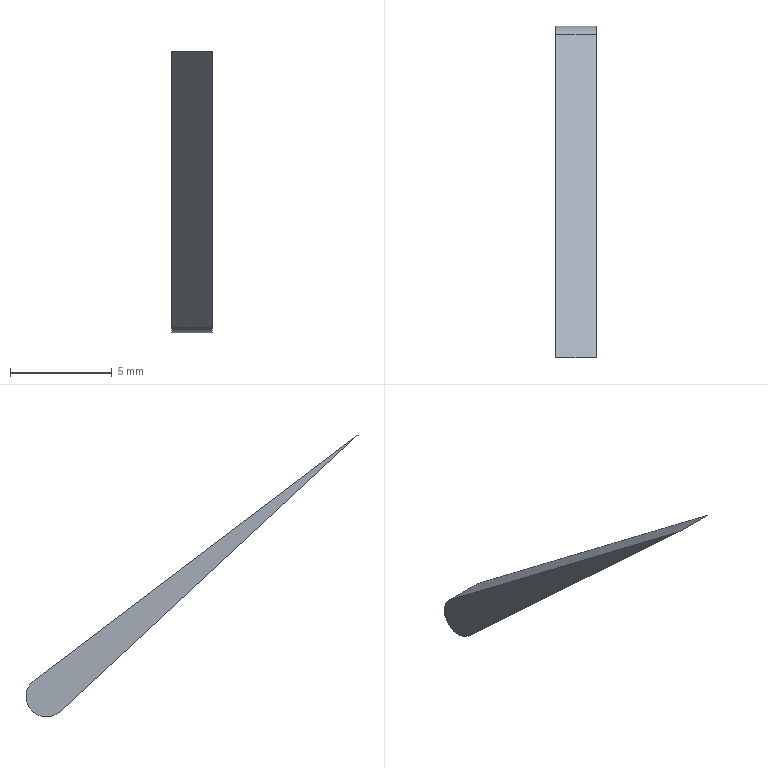Component | NX | SECONDHAND1 | 1 solid | 5 faces | box 2 x 16.32 x 13.86 mm | volume 43 mm3 | plane 4 | cylinder 1 | commonest cylinder face diameters 2 x1
STEP:
#1=CARTESIAN_POINT('',(0.,0.,0.));
#2=DIRECTION('',(0.,0.,1.));
#3=DIRECTION('',(1.,0.,0.));
#4=AXIS2_PLACEMENT_3D('',#1,#2,#3);
#5=CARTESIAN_POINT('',(-150.42,280.577,29.739));
#6=VERTEX_POINT('',#5);
#7=CARTESIAN_POINT('',(-150.42,281.861,31.269));
#8=VERTEX_POINT('',#7);
#9=CARTESIAN_POINT('',(-150.42,281.257,30.472));
#10=DIRECTION('',(1.,0.,0.));
#11=DIRECTION('',(0.,-0.766,0.6428));
#12=AXIS2_PLACEMENT_3D('',#9,#10,#11);
#13=CIRCLE('',#12,1.);
#14=CARTESIAN_POINT('',(-148.42,281.257,30.472));
#15=DIRECTION('',(-1.,0.,0.));
#16=DIRECTION('',(0.,0.766,-0.6428));
#17=AXIS2_PLACEMENT_3D('',#14,#15,#16);
#18=CYLINDRICAL_SURFACE('',#17,1.);
#19=CARTESIAN_POINT('',(9.425,2.));
#20=DIRECTION('',(-1.,0.));
#21=VECTOR('',#20,1.);
#22=LINE('',#19,#21);
#23=(GEOMETRIC_REPRESENTATION_CONTEXT(2)PARAMETRIC_REPRESENTATION_CONTEXT()REPRESENTATION_CONTEXT('',''));
#24=DEFINITIONAL_REPRESENTATION('',(#22),#23);
#25=PCURVE('',#18,#24);
#26=CARTESIAN_POINT('',(-150.42,281.257,30.472));
#27=DIRECTION('',(1.,0.,0.));
#28=DIRECTION('',(0.,-0.766,0.6428));
#29=AXIS2_PLACEMENT_3D('',#26,#27,#28);
#30=PLANE('',#29);
#31=CARTESIAN_POINT('',(0.,0.));
#32=DIRECTION('',(1.,-0.));
#33=AXIS2_PLACEMENT_2D('',#31,#32);
#34=CIRCLE('',#33,1.);
#35=(GEOMETRIC_REPRESENTATION_CONTEXT(2)PARAMETRIC_REPRESENTATION_CONTEXT()REPRESENTATION_CONTEXT('',''));
#36=DEFINITIONAL_REPRESENTATION('',(#34),#35);
#37=PCURVE('',#30,#36);
#38=SURFACE_CURVE('',#13,(#25,#37),.PCURVE_S1.);
#39=EDGE_CURVE('',#6,#8,#38,.T.);
#40=ORIENTED_EDGE('',*,*,#39,.T.);
#41=CARTESIAN_POINT('',(-148.42,281.861,31.269));
#42=VERTEX_POINT('',#41);
#43=CARTESIAN_POINT('',(-148.42,281.861,31.269));
#44=DIRECTION('',(-1.,0.,0.));
#45=VECTOR('',#44,1.);
#46=LINE('',#43,#45);
#47=CARTESIAN_POINT('',(4.662,0.));
#48=DIRECTION('',(0.,1.));
#49=VECTOR('',#48,1.);
#50=LINE('',#47,#49);
#51=(GEOMETRIC_REPRESENTATION_CONTEXT(2)PARAMETRIC_REPRESENTATION_CONTEXT()REPRESENTATION_CONTEXT('',''));
#52=DEFINITIONAL_REPRESENTATION('',(#50),#51);
#53=PCURVE('',#18,#52);
#54=CARTESIAN_POINT('',(-148.42,281.861,31.269));
#55=DIRECTION('',(0.,-0.6037,-0.7972));
#56=DIRECTION('',(0.,0.7972,-0.6037));
#57=AXIS2_PLACEMENT_3D('',#54,#55,#56);
#58=PLANE('',#57);
#59=CARTESIAN_POINT('',(-0.,0.));
#60=DIRECTION('',(0.,-1.));
#61=VECTOR('',#60,1.);
#62=LINE('',#59,#61);
#63=(GEOMETRIC_REPRESENTATION_CONTEXT(2)PARAMETRIC_REPRESENTATION_CONTEXT()REPRESENTATION_CONTEXT('',''));
#64=DEFINITIONAL_REPRESENTATION('',(#62),#63);
#65=PCURVE('',#58,#64);
#66=SURFACE_CURVE('',#46,(#53,#65),.PCURVE_S1.);
#67=EDGE_CURVE('',#42,#8,#66,.T.);
#68=ORIENTED_EDGE('',*,*,#67,.F.);
#69=CARTESIAN_POINT('',(-148.42,280.577,29.739));
#70=VERTEX_POINT('',#69);
#71=CARTESIAN_POINT('',(-148.42,281.257,30.472));
#72=DIRECTION('',(1.,0.,0.));
#73=DIRECTION('',(0.,-0.766,0.6428));
#74=AXIS2_PLACEMENT_3D('',#71,#72,#73);
#75=CIRCLE('',#74,1.);
#76=CARTESIAN_POINT('',(9.425,0.));
#77=DIRECTION('',(-1.,0.));
#78=VECTOR('',#77,1.);
#79=LINE('',#76,#78);
#80=(GEOMETRIC_REPRESENTATION_CONTEXT(2)PARAMETRIC_REPRESENTATION_CONTEXT()REPRESENTATION_CONTEXT('',''));
#81=DEFINITIONAL_REPRESENTATION('',(#79),#80);
#82=PCURVE('',#18,#81);
#83=CARTESIAN_POINT('',(-148.42,281.257,30.472));
#84=DIRECTION('',(1.,0.,0.));
#85=DIRECTION('',(0.,-0.766,0.6428));
#86=AXIS2_PLACEMENT_3D('',#83,#84,#85);
#87=PLANE('',#86);
#88=CARTESIAN_POINT('',(0.,0.));
#89=DIRECTION('',(1.,-0.));
#90=AXIS2_PLACEMENT_2D('',#88,#89);
#91=CIRCLE('',#90,1.);
#92=(GEOMETRIC_REPRESENTATION_CONTEXT(2)PARAMETRIC_REPRESENTATION_CONTEXT()REPRESENTATION_CONTEXT('',''));
#93=DEFINITIONAL_REPRESENTATION('',(#91),#92);
#94=PCURVE('',#87,#93);
#95=SURFACE_CURVE('',#75,(#82,#94),.PCURVE_S1.);
#96=EDGE_CURVE('',#70,#42,#95,.T.);
#97=ORIENTED_EDGE('',*,*,#96,.F.);
#98=CARTESIAN_POINT('',(-148.42,280.577,29.739));
#99=DIRECTION('',(-1.,0.,0.));
#100=VECTOR('',#99,1.);
#101=LINE('',#98,#100);
#102=CARTESIAN_POINT('',(7.904,0.));
#103=DIRECTION('',(0.,1.));
#104=VECTOR('',#103,1.);
#105=LINE('',#102,#104);
#106=(GEOMETRIC_REPRESENTATION_CONTEXT(2)PARAMETRIC_REPRESENTATION_CONTEXT()REPRESENTATION_CONTEXT('',''));
#107=DEFINITIONAL_REPRESENTATION('',(#105),#106);
#108=PCURVE('',#18,#107);
#109=CARTESIAN_POINT('',(-148.42,265.936,43.327));
#110=DIRECTION('',(0.,0.6803,0.7329));
#111=DIRECTION('',(0.,-0.7329,0.6803));
#112=AXIS2_PLACEMENT_3D('',#109,#110,#111);
#113=PLANE('',#112);
#114=CARTESIAN_POINT('',(-19.975,0.));
#115=DIRECTION('',(0.,-1.));
#116=VECTOR('',#115,1.);
#117=LINE('',#114,#116);
#118=(GEOMETRIC_REPRESENTATION_CONTEXT(2)PARAMETRIC_REPRESENTATION_CONTEXT()REPRESENTATION_CONTEXT('',''));
#119=DEFINITIONAL_REPRESENTATION('',(#117),#118);
#120=PCURVE('',#113,#119);
#121=SURFACE_CURVE('',#101,(#108,#120),.PCURVE_S1.);
#122=EDGE_CURVE('',#70,#6,#121,.T.);
#123=ORIENTED_EDGE('',*,*,#122,.T.);
#124=EDGE_LOOP('',(#40,#68,#97,#123));
#125=FACE_BOUND('',#124,.T.);
#126=ADVANCED_FACE('',(#125),#18,.T.);
#127=CARTESIAN_POINT('',(-150.42,265.936,43.327));
#128=VERTEX_POINT('',#127);
#129=CARTESIAN_POINT('',(-150.42,281.861,31.269));
#130=DIRECTION('',(0.,-0.7972,0.6037));
#131=VECTOR('',#130,1.);
#132=LINE('',#129,#131);
#133=CARTESIAN_POINT('',(0.,-2.));
#134=DIRECTION('',(-1.,0.));
#135=VECTOR('',#134,1.);
#136=LINE('',#133,#135);
#137=(GEOMETRIC_REPRESENTATION_CONTEXT(2)PARAMETRIC_REPRESENTATION_CONTEXT()REPRESENTATION_CONTEXT('',''));
#138=DEFINITIONAL_REPRESENTATION('',(#136),#137);
#139=PCURVE('',#58,#138);
#140=CARTESIAN_POINT('',(0.05,-0.9987));
#141=DIRECTION('',(0.9987,0.05));
#142=VECTOR('',#141,1.);
#143=LINE('',#140,#142);
#144=(GEOMETRIC_REPRESENTATION_CONTEXT(2)PARAMETRIC_REPRESENTATION_CONTEXT()REPRESENTATION_CONTEXT('',''));
#145=DEFINITIONAL_REPRESENTATION('',(#143),#144);
#146=PCURVE('',#30,#145);
#147=SURFACE_CURVE('',#132,(#139,#146),.PCURVE_S1.);
#148=EDGE_CURVE('',#8,#128,#147,.T.);
#149=ORIENTED_EDGE('',*,*,#148,.T.);
#150=CARTESIAN_POINT('',(-148.42,265.936,43.327));
#151=VERTEX_POINT('',#150);
#152=CARTESIAN_POINT('',(-148.42,265.936,43.327));
#153=DIRECTION('',(-1.,0.,0.));
#154=VECTOR('',#153,1.);
#155=LINE('',#152,#154);
#156=CARTESIAN_POINT('',(-19.975,0.));
#157=DIRECTION('',(0.,-1.));
#158=VECTOR('',#157,1.);
#159=LINE('',#156,#158);
#160=(GEOMETRIC_REPRESENTATION_CONTEXT(2)PARAMETRIC_REPRESENTATION_CONTEXT()REPRESENTATION_CONTEXT('',''));
#161=DEFINITIONAL_REPRESENTATION('',(#159),#160);
#162=PCURVE('',#58,#161);
#163=CARTESIAN_POINT('',(0.,0.));
#164=DIRECTION('',(0.,-1.));
#165=VECTOR('',#164,1.);
#166=LINE('',#163,#165);
#167=(GEOMETRIC_REPRESENTATION_CONTEXT(2)PARAMETRIC_REPRESENTATION_CONTEXT()REPRESENTATION_CONTEXT('',''));
#168=DEFINITIONAL_REPRESENTATION('',(#166),#167);
#169=PCURVE('',#113,#168);
#170=SURFACE_CURVE('',#155,(#162,#169),.PCURVE_S1.);
#171=EDGE_CURVE('',#151,#128,#170,.T.);
#172=ORIENTED_EDGE('',*,*,#171,.F.);
#173=CARTESIAN_POINT('',(-148.42,281.861,31.269));
#174=DIRECTION('',(0.,-0.7972,0.6037));
#175=VECTOR('',#174,1.);
#176=LINE('',#173,#175);
#177=CARTESIAN_POINT('',(0.,0.));
#178=DIRECTION('',(-1.,0.));
#179=VECTOR('',#178,1.);
#180=LINE('',#177,#179);
#181=(GEOMETRIC_REPRESENTATION_CONTEXT(2)PARAMETRIC_REPRESENTATION_CONTEXT()REPRESENTATION_CONTEXT('',''));
#182=DEFINITIONAL_REPRESENTATION('',(#180),#181);
#183=PCURVE('',#58,#182);
#184=CARTESIAN_POINT('',(0.05,-0.9987));
#185=DIRECTION('',(0.9987,0.05));
#186=VECTOR('',#185,1.);
#187=LINE('',#184,#186);
#188=(GEOMETRIC_REPRESENTATION_CONTEXT(2)PARAMETRIC_REPRESENTATION_CONTEXT()REPRESENTATION_CONTEXT('',''));
#189=DEFINITIONAL_REPRESENTATION('',(#187),#188);
#190=PCURVE('',#87,#189);
#191=SURFACE_CURVE('',#176,(#183,#190),.PCURVE_S1.);
#192=EDGE_CURVE('',#42,#151,#191,.T.);
#193=ORIENTED_EDGE('',*,*,#192,.F.);
#194=ORIENTED_EDGE('',*,*,#67,.T.);
#195=EDGE_LOOP('',(#149,#172,#193,#194));
#196=FACE_BOUND('',#195,.T.);
#197=ADVANCED_FACE('',(#196),#58,.F.);
#198=CARTESIAN_POINT('',(-150.42,265.936,43.327));
#199=DIRECTION('',(0.,0.7329,-0.6803));
#200=VECTOR('',#199,1.);
#201=LINE('',#198,#200);
#202=CARTESIAN_POINT('',(0.,-2.));
#203=DIRECTION('',(-1.,0.));
#204=VECTOR('',#203,1.);
#205=LINE('',#202,#204);
#206=(GEOMETRIC_REPRESENTATION_CONTEXT(2)PARAMETRIC_REPRESENTATION_CONTEXT()REPRESENTATION_CONTEXT('',''));
#207=DEFINITIONAL_REPRESENTATION('',(#205),#206);
#208=PCURVE('',#113,#207);
#209=CARTESIAN_POINT('',(20.,0.));
#210=DIRECTION('',(-0.9987,0.05));
#211=VECTOR('',#210,1.);
#212=LINE('',#209,#211);
#213=(GEOMETRIC_REPRESENTATION_CONTEXT(2)PARAMETRIC_REPRESENTATION_CONTEXT()REPRESENTATION_CONTEXT('',''));
#214=DEFINITIONAL_REPRESENTATION('',(#212),#213);
#215=PCURVE('',#30,#214);
#216=SURFACE_CURVE('',#201,(#208,#215),.PCURVE_S1.);
#217=EDGE_CURVE('',#128,#6,#216,.T.);
#218=ORIENTED_EDGE('',*,*,#217,.T.);
#219=ORIENTED_EDGE('',*,*,#122,.F.);
#220=CARTESIAN_POINT('',(-148.42,265.936,43.327));
#221=DIRECTION('',(0.,0.7329,-0.6803));
#222=VECTOR('',#221,1.);
#223=LINE('',#220,#222);
#224=CARTESIAN_POINT('',(0.,0.));
#225=DIRECTION('',(-1.,0.));
#226=VECTOR('',#225,1.);
#227=LINE('',#224,#226);
#228=(GEOMETRIC_REPRESENTATION_CONTEXT(2)PARAMETRIC_REPRESENTATION_CONTEXT()REPRESENTATION_CONTEXT('',''));
#229=DEFINITIONAL_REPRESENTATION('',(#227),#228);
#230=PCURVE('',#113,#229);
#231=CARTESIAN_POINT('',(20.,0.));
#232=DIRECTION('',(-0.9987,0.05));
#233=VECTOR('',#232,1.);
#234=LINE('',#231,#233);
#235=(GEOMETRIC_REPRESENTATION_CONTEXT(2)PARAMETRIC_REPRESENTATION_CONTEXT()REPRESENTATION_CONTEXT('',''));
#236=DEFINITIONAL_REPRESENTATION('',(#234),#235);
#237=PCURVE('',#87,#236);
#238=SURFACE_CURVE('',#223,(#230,#237),.PCURVE_S1.);
#239=EDGE_CURVE('',#151,#70,#238,.T.);
#240=ORIENTED_EDGE('',*,*,#239,.F.);
#241=ORIENTED_EDGE('',*,*,#171,.T.);
#242=EDGE_LOOP('',(#218,#219,#240,#241));
#243=FACE_BOUND('',#242,.T.);
#244=ADVANCED_FACE('',(#243),#113,.F.);
#245=ORIENTED_EDGE('',*,*,#96,.T.);
#246=ORIENTED_EDGE('',*,*,#192,.T.);
#247=ORIENTED_EDGE('',*,*,#239,.T.);
#248=EDGE_LOOP('',(#245,#246,#247));
#249=FACE_BOUND('',#248,.T.);
#250=ADVANCED_FACE('',(#249),#87,.T.);
#251=ORIENTED_EDGE('',*,*,#39,.F.);
#252=ORIENTED_EDGE('',*,*,#217,.F.);
#253=ORIENTED_EDGE('',*,*,#148,.F.);
#254=EDGE_LOOP('',(#251,#252,#253));
#255=FACE_BOUND('',#254,.T.);
#256=ADVANCED_FACE('',(#255),#30,.F.);
#257=CLOSED_SHELL('',(#126,#197,#244,#250,#256));
#258=MANIFOLD_SOLID_BREP('',#257);
#259=(LENGTH_UNIT()NAMED_UNIT(*)SI_UNIT(.MILLI.,.METRE.));
#260=UNCERTAINTY_MEASURE_WITH_UNIT(LENGTH_MEASURE(0.0000001),#259,'','');
#261=(NAMED_UNIT(*)PLANE_ANGLE_UNIT()SI_UNIT($,.RADIAN.));
#262=(NAMED_UNIT(*)SI_UNIT($,.STERADIAN.)SOLID_ANGLE_UNIT());
#263=(GEOMETRIC_REPRESENTATION_CONTEXT(3)GLOBAL_UNCERTAINTY_ASSIGNED_CONTEXT((#260))GLOBAL_UNIT_ASSIGNED_CONTEXT((#259,#261,#262))REPRESENTATION_CONTEXT('',''));
#264=ADVANCED_BREP_SHAPE_REPRESENTATION('',(#4,#258),#263);